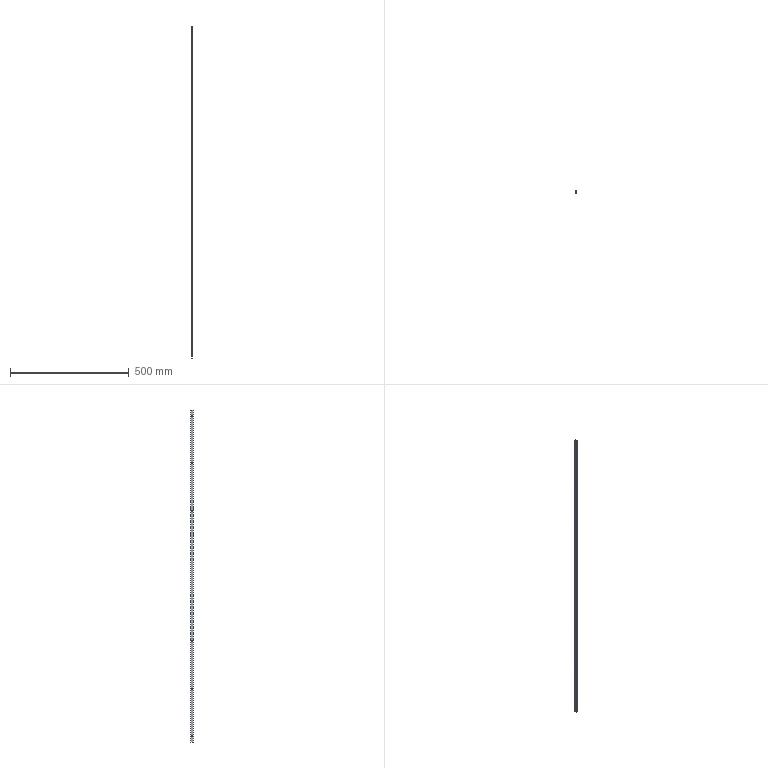Component | SolidWorks | GroundingSystem-1_GroundingCopperBar-1 | 1 solid | 18 faces | box 4 x 12 x 1400 mm | volume 66952 mm3 | cylinder 12 | plane 6 | commonest cylinder face diameters 3.3 x8 4.2 x4
STEP:
#1=COLOUR_RGB('',0.7922,0.8196,0.9333);
#2=FILL_AREA_STYLE_COLOUR('',#1);
#3=FILL_AREA_STYLE('',(#2));
#4=SURFACE_STYLE_FILL_AREA(#3);
#5=SURFACE_SIDE_STYLE('',(#4));
#6=SURFACE_STYLE_USAGE(.BOTH.,#5);
#7=PRESENTATION_STYLE_ASSIGNMENT((#6));
#8=CARTESIAN_POINT('',(10.505,-0.4112,58.688));
#9=VERTEX_POINT('',#8);
#10=CARTESIAN_POINT('',(10.505,-0.4112,58.853));
#11=VERTEX_POINT('',#10);
#12=CARTESIAN_POINT('',(10.505,-0.4112,58.771));
#13=DIRECTION('',(1.,0.,-0.));
#14=DIRECTION('',(0.,0.,1.));
#15=AXIS2_PLACEMENT_3D('',#12,#13,#14);
#16=CIRCLE('',#15,0.08268);
#17=EDGE_CURVE('',#9,#11,#16,.T.);
#18=ORIENTED_EDGE('',*,*,#17,.T.);
#19=CARTESIAN_POINT('',(10.348,-0.4112,58.853));
#20=VERTEX_POINT('',#19);
#21=CARTESIAN_POINT('',(10.348,-0.4112,58.853));
#22=DIRECTION('',(-1.,-0.,0.));
#23=VECTOR('',#22,39.37);
#24=LINE('',#21,#23);
#25=EDGE_CURVE('',#11,#20,#24,.T.);
#26=ORIENTED_EDGE('',*,*,#25,.T.);
#27=CARTESIAN_POINT('',(10.348,-0.4112,58.688));
#28=VERTEX_POINT('',#27);
#29=CARTESIAN_POINT('',(10.348,-0.4112,58.771));
#30=DIRECTION('',(-1.,-0.,0.));
#31=DIRECTION('',(0.,-0.,-1.));
#32=AXIS2_PLACEMENT_3D('',#29,#30,#31);
#33=CIRCLE('',#32,0.08268);
#34=EDGE_CURVE('',#20,#28,#33,.T.);
#35=ORIENTED_EDGE('',*,*,#34,.T.);
#36=CARTESIAN_POINT('',(10.348,-0.4112,58.688));
#37=DIRECTION('',(-1.,-0.,0.));
#38=VECTOR('',#37,39.37);
#39=LINE('',#36,#38);
#40=EDGE_CURVE('',#9,#28,#39,.T.);
#41=ORIENTED_EDGE('',*,*,#40,.F.);
#42=EDGE_LOOP('',(#18,#26,#35,#41));
#43=FACE_OUTER_BOUND('',#42,.T.);
#44=CARTESIAN_POINT('',(10.348,-0.4112,58.771));
#45=DIRECTION('',(-1.,-0.,0.));
#46=DIRECTION('',(0.,-0.,-1.));
#47=AXIS2_PLACEMENT_3D('',#44,#45,#46);
#48=CYLINDRICAL_SURFACE('',#47,0.08268);
#49=ADVANCED_FACE('',(#43),#48,.F.);
#50=CARTESIAN_POINT('',(10.505,-0.4112,5.538));
#51=VERTEX_POINT('',#50);
#52=CARTESIAN_POINT('',(10.505,-0.4112,5.704));
#53=VERTEX_POINT('',#52);
#54=CARTESIAN_POINT('',(10.505,-0.4112,5.621));
#55=DIRECTION('',(1.,0.,-0.));
#56=DIRECTION('',(0.,0.,1.));
#57=AXIS2_PLACEMENT_3D('',#54,#55,#56);
#58=CIRCLE('',#57,0.08268);
#59=EDGE_CURVE('',#51,#53,#58,.T.);
#60=ORIENTED_EDGE('',*,*,#59,.T.);
#61=CARTESIAN_POINT('',(10.348,-0.4112,5.704));
#62=VERTEX_POINT('',#61);
#63=CARTESIAN_POINT('',(10.348,-0.4112,5.704));
#64=DIRECTION('',(-1.,-0.,0.));
#65=VECTOR('',#64,39.37);
#66=LINE('',#63,#65);
#67=EDGE_CURVE('',#53,#62,#66,.T.);
#68=ORIENTED_EDGE('',*,*,#67,.T.);
#69=CARTESIAN_POINT('',(10.348,-0.4112,5.538));
#70=VERTEX_POINT('',#69);
#71=CARTESIAN_POINT('',(10.348,-0.4112,5.621));
#72=DIRECTION('',(-1.,-0.,0.));
#73=DIRECTION('',(0.,-0.,-1.));
#74=AXIS2_PLACEMENT_3D('',#71,#72,#73);
#75=CIRCLE('',#74,0.08268);
#76=EDGE_CURVE('',#62,#70,#75,.T.);
#77=ORIENTED_EDGE('',*,*,#76,.T.);
#78=CARTESIAN_POINT('',(10.348,-0.4112,5.538));
#79=DIRECTION('',(-1.,-0.,0.));
#80=VECTOR('',#79,39.37);
#81=LINE('',#78,#80);
#82=EDGE_CURVE('',#51,#70,#81,.T.);
#83=ORIENTED_EDGE('',*,*,#82,.F.);
#84=EDGE_LOOP('',(#60,#68,#77,#83));
#85=FACE_OUTER_BOUND('',#84,.T.);
#86=CARTESIAN_POINT('',(10.348,-0.4112,5.621));
#87=DIRECTION('',(-1.,-0.,0.));
#88=DIRECTION('',(0.,-0.,-1.));
#89=AXIS2_PLACEMENT_3D('',#86,#87,#88);
#90=CYLINDRICAL_SURFACE('',#89,0.08268);
#91=ADVANCED_FACE('',(#85),#90,.F.);
#92=CARTESIAN_POINT('',(10.505,-0.4112,50.832));
#93=VERTEX_POINT('',#92);
#94=CARTESIAN_POINT('',(10.505,-0.4112,50.962));
#95=VERTEX_POINT('',#94);
#96=CARTESIAN_POINT('',(10.505,-0.4112,50.897));
#97=DIRECTION('',(1.,0.,-0.));
#98=DIRECTION('',(0.,0.,1.));
#99=AXIS2_PLACEMENT_3D('',#96,#97,#98);
#100=CIRCLE('',#99,0.06496);
#101=EDGE_CURVE('',#93,#95,#100,.T.);
#102=ORIENTED_EDGE('',*,*,#101,.T.);
#103=CARTESIAN_POINT('',(10.348,-0.4112,50.962));
#104=VERTEX_POINT('',#103);
#105=CARTESIAN_POINT('',(10.348,-0.4112,50.962));
#106=DIRECTION('',(-1.,-0.,0.));
#107=VECTOR('',#106,39.37);
#108=LINE('',#105,#107);
#109=EDGE_CURVE('',#95,#104,#108,.T.);
#110=ORIENTED_EDGE('',*,*,#109,.T.);
#111=CARTESIAN_POINT('',(10.348,-0.4112,50.832));
#112=VERTEX_POINT('',#111);
#113=CARTESIAN_POINT('',(10.348,-0.4112,50.897));
#114=DIRECTION('',(-1.,-0.,0.));
#115=DIRECTION('',(0.,-0.,-1.));
#116=AXIS2_PLACEMENT_3D('',#113,#114,#115);
#117=CIRCLE('',#116,0.06496);
#118=EDGE_CURVE('',#104,#112,#117,.T.);
#119=ORIENTED_EDGE('',*,*,#118,.T.);
#120=CARTESIAN_POINT('',(10.348,-0.4112,50.832));
#121=DIRECTION('',(-1.,-0.,0.));
#122=VECTOR('',#121,39.37);
#123=LINE('',#120,#122);
#124=EDGE_CURVE('',#93,#112,#123,.T.);
#125=ORIENTED_EDGE('',*,*,#124,.F.);
#126=EDGE_LOOP('',(#102,#110,#119,#125));
#127=FACE_OUTER_BOUND('',#126,.T.);
#128=CARTESIAN_POINT('',(10.348,-0.4112,50.897));
#129=DIRECTION('',(-1.,-0.,0.));
#130=DIRECTION('',(0.,-0.,-1.));
#131=AXIS2_PLACEMENT_3D('',#128,#129,#130);
#132=CYLINDRICAL_SURFACE('',#131,0.06496);
#133=ADVANCED_FACE('',(#127),#132,.F.);
#134=CARTESIAN_POINT('',(10.505,-0.4112,42.958));
#135=VERTEX_POINT('',#134);
#136=CARTESIAN_POINT('',(10.505,-0.4112,43.088));
#137=VERTEX_POINT('',#136);
#138=CARTESIAN_POINT('',(10.505,-0.4112,43.023));
#139=DIRECTION('',(1.,0.,-0.));
#140=DIRECTION('',(0.,0.,1.));
#141=AXIS2_PLACEMENT_3D('',#138,#139,#140);
#142=CIRCLE('',#141,0.06496);
#143=EDGE_CURVE('',#135,#137,#142,.T.);
#144=ORIENTED_EDGE('',*,*,#143,.T.);
#145=CARTESIAN_POINT('',(10.348,-0.4112,43.088));
#146=VERTEX_POINT('',#145);
#147=CARTESIAN_POINT('',(10.348,-0.4112,43.088));
#148=DIRECTION('',(-1.,-0.,0.));
#149=VECTOR('',#148,39.37);
#150=LINE('',#147,#149);
#151=EDGE_CURVE('',#137,#146,#150,.T.);
#152=ORIENTED_EDGE('',*,*,#151,.T.);
#153=CARTESIAN_POINT('',(10.348,-0.4112,42.958));
#154=VERTEX_POINT('',#153);
#155=CARTESIAN_POINT('',(10.348,-0.4112,43.023));
#156=DIRECTION('',(-1.,-0.,0.));
#157=DIRECTION('',(0.,-0.,-1.));
#158=AXIS2_PLACEMENT_3D('',#155,#156,#157);
#159=CIRCLE('',#158,0.06496);
#160=EDGE_CURVE('',#146,#154,#159,.T.);
#161=ORIENTED_EDGE('',*,*,#160,.T.);
#162=CARTESIAN_POINT('',(10.348,-0.4112,42.958));
#163=DIRECTION('',(-1.,-0.,0.));
#164=VECTOR('',#163,39.37);
#165=LINE('',#162,#164);
#166=EDGE_CURVE('',#135,#154,#165,.T.);
#167=ORIENTED_EDGE('',*,*,#166,.F.);
#168=EDGE_LOOP('',(#144,#152,#161,#167));
#169=FACE_OUTER_BOUND('',#168,.T.);
#170=CARTESIAN_POINT('',(10.348,-0.4112,43.023));
#171=DIRECTION('',(-1.,-0.,0.));
#172=DIRECTION('',(0.,-0.,-1.));
#173=AXIS2_PLACEMENT_3D('',#170,#171,#172);
#174=CYLINDRICAL_SURFACE('',#173,0.06496);
#175=ADVANCED_FACE('',(#169),#174,.F.);
#176=CARTESIAN_POINT('',(10.505,-0.4112,13.43));
#177=VERTEX_POINT('',#176);
#178=CARTESIAN_POINT('',(10.505,-0.4112,13.56));
#179=VERTEX_POINT('',#178);
#180=CARTESIAN_POINT('',(10.505,-0.4112,13.495));
#181=DIRECTION('',(1.,0.,-0.));
#182=DIRECTION('',(0.,0.,1.));
#183=AXIS2_PLACEMENT_3D('',#180,#181,#182);
#184=CIRCLE('',#183,0.06496);
#185=EDGE_CURVE('',#177,#179,#184,.T.);
#186=ORIENTED_EDGE('',*,*,#185,.T.);
#187=CARTESIAN_POINT('',(10.348,-0.4112,13.56));
#188=VERTEX_POINT('',#187);
#189=CARTESIAN_POINT('',(10.348,-0.4112,13.56));
#190=DIRECTION('',(-1.,-0.,0.));
#191=VECTOR('',#190,39.37);
#192=LINE('',#189,#191);
#193=EDGE_CURVE('',#179,#188,#192,.T.);
#194=ORIENTED_EDGE('',*,*,#193,.T.);
#195=CARTESIAN_POINT('',(10.348,-0.4112,13.43));
#196=VERTEX_POINT('',#195);
#197=CARTESIAN_POINT('',(10.348,-0.4112,13.495));
#198=DIRECTION('',(-1.,-0.,0.));
#199=DIRECTION('',(0.,-0.,-1.));
#200=AXIS2_PLACEMENT_3D('',#197,#198,#199);
#201=CIRCLE('',#200,0.06496);
#202=EDGE_CURVE('',#188,#196,#201,.T.);
#203=ORIENTED_EDGE('',*,*,#202,.T.);
#204=CARTESIAN_POINT('',(10.348,-0.4112,13.43));
#205=DIRECTION('',(-1.,-0.,0.));
#206=VECTOR('',#205,39.37);
#207=LINE('',#204,#206);
#208=EDGE_CURVE('',#177,#196,#207,.T.);
#209=ORIENTED_EDGE('',*,*,#208,.F.);
#210=EDGE_LOOP('',(#186,#194,#203,#209));
#211=FACE_OUTER_BOUND('',#210,.T.);
#212=CARTESIAN_POINT('',(10.348,-0.4112,13.495));
#213=DIRECTION('',(-1.,-0.,0.));
#214=DIRECTION('',(0.,-0.,-1.));
#215=AXIS2_PLACEMENT_3D('',#212,#213,#214);
#216=CYLINDRICAL_SURFACE('',#215,0.06496);
#217=ADVANCED_FACE('',(#211),#216,.F.);
#218=CARTESIAN_POINT('',(10.505,-0.4112,21.304));
#219=VERTEX_POINT('',#218);
#220=CARTESIAN_POINT('',(10.505,-0.4112,21.434));
#221=VERTEX_POINT('',#220);
#222=CARTESIAN_POINT('',(10.505,-0.4112,21.369));
#223=DIRECTION('',(1.,0.,-0.));
#224=DIRECTION('',(0.,0.,1.));
#225=AXIS2_PLACEMENT_3D('',#222,#223,#224);
#226=CIRCLE('',#225,0.06496);
#227=EDGE_CURVE('',#219,#221,#226,.T.);
#228=ORIENTED_EDGE('',*,*,#227,.T.);
#229=CARTESIAN_POINT('',(10.348,-0.4112,21.434));
#230=VERTEX_POINT('',#229);
#231=CARTESIAN_POINT('',(10.348,-0.4112,21.434));
#232=DIRECTION('',(-1.,-0.,0.));
#233=VECTOR('',#232,39.37);
#234=LINE('',#231,#233);
#235=EDGE_CURVE('',#221,#230,#234,.T.);
#236=ORIENTED_EDGE('',*,*,#235,.T.);
#237=CARTESIAN_POINT('',(10.348,-0.4112,21.304));
#238=VERTEX_POINT('',#237);
#239=CARTESIAN_POINT('',(10.348,-0.4112,21.369));
#240=DIRECTION('',(-1.,-0.,0.));
#241=DIRECTION('',(0.,-0.,-1.));
#242=AXIS2_PLACEMENT_3D('',#239,#240,#241);
#243=CIRCLE('',#242,0.06496);
#244=EDGE_CURVE('',#230,#238,#243,.T.);
#245=ORIENTED_EDGE('',*,*,#244,.T.);
#246=CARTESIAN_POINT('',(10.348,-0.4112,21.304));
#247=DIRECTION('',(-1.,-0.,0.));
#248=VECTOR('',#247,39.37);
#249=LINE('',#246,#248);
#250=EDGE_CURVE('',#219,#238,#249,.T.);
#251=ORIENTED_EDGE('',*,*,#250,.F.);
#252=EDGE_LOOP('',(#228,#236,#245,#251));
#253=FACE_OUTER_BOUND('',#252,.T.);
#254=CARTESIAN_POINT('',(10.348,-0.4112,21.369));
#255=DIRECTION('',(-1.,-0.,0.));
#256=DIRECTION('',(0.,-0.,-1.));
#257=AXIS2_PLACEMENT_3D('',#254,#255,#256);
#258=CYLINDRICAL_SURFACE('',#257,0.06496);
#259=ADVANCED_FACE('',(#253),#258,.F.);
#260=CARTESIAN_POINT('',(10.348,-0.175,4.637));
#261=VERTEX_POINT('',#260);
#262=CARTESIAN_POINT('',(10.348,-0.6474,4.637));
#263=VERTEX_POINT('',#262);
#264=CARTESIAN_POINT('',(10.348,-0.175,4.637));
#265=DIRECTION('',(0.,-1.,0.));
#266=VECTOR('',#265,39.37);
#267=LINE('',#264,#266);
#268=EDGE_CURVE('',#261,#263,#267,.T.);
#269=ORIENTED_EDGE('',*,*,#268,.F.);
#270=CARTESIAN_POINT('',(10.505,-0.175,4.637));
#271=VERTEX_POINT('',#270);
#272=CARTESIAN_POINT('',(10.505,-0.175,4.637));
#273=DIRECTION('',(-1.,-0.,0.));
#274=VECTOR('',#273,39.37);
#275=LINE('',#272,#274);
#276=EDGE_CURVE('',#271,#261,#275,.T.);
#277=ORIENTED_EDGE('',*,*,#276,.F.);
#278=CARTESIAN_POINT('',(10.505,-0.6474,4.637));
#279=VERTEX_POINT('',#278);
#280=CARTESIAN_POINT('',(10.505,-0.175,4.637));
#281=DIRECTION('',(0.,-1.,0.));
#282=VECTOR('',#281,39.37);
#283=LINE('',#280,#282);
#284=EDGE_CURVE('',#271,#279,#283,.T.);
#285=ORIENTED_EDGE('',*,*,#284,.T.);
#286=CARTESIAN_POINT('',(10.505,-0.6474,4.637));
#287=DIRECTION('',(-1.,-0.,0.));
#288=VECTOR('',#287,39.37);
#289=LINE('',#286,#288);
#290=EDGE_CURVE('',#279,#263,#289,.T.);
#291=ORIENTED_EDGE('',*,*,#290,.T.);
#292=EDGE_LOOP('',(#269,#277,#285,#291));
#293=FACE_OUTER_BOUND('',#292,.T.);
#294=CARTESIAN_POINT('',(10.505,-0.175,4.637));
#295=DIRECTION('',(-0.,-0.,-1.));
#296=DIRECTION('',(1.,0.,-0.));
#297=AXIS2_PLACEMENT_3D('',#294,#295,#296);
#298=PLANE('',#297);
#299=ADVANCED_FACE('',(#293),#298,.T.);
#300=CARTESIAN_POINT('',(10.348,-0.175,59.755));
#301=VERTEX_POINT('',#300);
#302=CARTESIAN_POINT('',(10.348,-0.175,59.755));
#303=DIRECTION('',(-0.,-0.,-1.));
#304=VECTOR('',#303,39.37);
#305=LINE('',#302,#304);
#306=EDGE_CURVE('',#301,#261,#305,.T.);
#307=ORIENTED_EDGE('',*,*,#306,.F.);
#308=CARTESIAN_POINT('',(10.505,-0.175,59.755));
#309=VERTEX_POINT('',#308);
#310=CARTESIAN_POINT('',(10.505,-0.175,59.755));
#311=DIRECTION('',(-1.,-0.,0.));
#312=VECTOR('',#311,39.37);
#313=LINE('',#310,#312);
#314=EDGE_CURVE('',#309,#301,#313,.T.);
#315=ORIENTED_EDGE('',*,*,#314,.F.);
#316=CARTESIAN_POINT('',(10.505,-0.175,59.755));
#317=DIRECTION('',(-0.,-0.,-1.));
#318=VECTOR('',#317,39.37);
#319=LINE('',#316,#318);
#320=EDGE_CURVE('',#309,#271,#319,.T.);
#321=ORIENTED_EDGE('',*,*,#320,.T.);
#322=ORIENTED_EDGE('',*,*,#276,.T.);
#323=EDGE_LOOP('',(#307,#315,#321,#322));
#324=FACE_OUTER_BOUND('',#323,.T.);
#325=CARTESIAN_POINT('',(10.505,-0.175,59.755));
#326=DIRECTION('',(-0.,1.,-0.));
#327=DIRECTION('',(1.,0.,-0.));
#328=AXIS2_PLACEMENT_3D('',#325,#326,#327);
#329=PLANE('',#328);
#330=ADVANCED_FACE('',(#324),#329,.T.);
#331=CARTESIAN_POINT('',(10.348,-0.6474,59.755));
#332=VERTEX_POINT('',#331);
#333=CARTESIAN_POINT('',(10.348,-0.175,59.755));
#334=DIRECTION('',(-0.,1.,-0.));
#335=VECTOR('',#334,39.37);
#336=LINE('',#333,#335);
#337=EDGE_CURVE('',#332,#301,#336,.T.);
#338=ORIENTED_EDGE('',*,*,#337,.F.);
#339=CARTESIAN_POINT('',(10.505,-0.6474,59.755));
#340=VERTEX_POINT('',#339);
#341=CARTESIAN_POINT('',(10.505,-0.6474,59.755));
#342=DIRECTION('',(-1.,-0.,0.));
#343=VECTOR('',#342,39.37);
#344=LINE('',#341,#343);
#345=EDGE_CURVE('',#340,#332,#344,.T.);
#346=ORIENTED_EDGE('',*,*,#345,.F.);
#347=CARTESIAN_POINT('',(10.505,-0.175,59.755));
#348=DIRECTION('',(-0.,1.,-0.));
#349=VECTOR('',#348,39.37);
#350=LINE('',#347,#349);
#351=EDGE_CURVE('',#340,#309,#350,.T.);
#352=ORIENTED_EDGE('',*,*,#351,.T.);
#353=ORIENTED_EDGE('',*,*,#314,.T.);
#354=EDGE_LOOP('',(#338,#346,#352,#353));
#355=FACE_OUTER_BOUND('',#354,.T.);
#356=CARTESIAN_POINT('',(10.505,-0.175,59.755));
#357=DIRECTION('',(0.,0.,1.));
#358=DIRECTION('',(-1.,-0.,0.));
#359=AXIS2_PLACEMENT_3D('',#356,#357,#358);
#360=PLANE('',#359);
#361=ADVANCED_FACE('',(#355),#360,.T.);
#362=CARTESIAN_POINT('',(10.348,-0.6474,59.755));
#363=DIRECTION('',(0.,0.,1.));
#364=VECTOR('',#363,39.37);
#365=LINE('',#362,#364);
#366=EDGE_CURVE('',#263,#332,#365,.T.);
#367=ORIENTED_EDGE('',*,*,#366,.F.);
#368=ORIENTED_EDGE('',*,*,#290,.F.);
#369=CARTESIAN_POINT('',(10.505,-0.6474,59.755));
#370=DIRECTION('',(0.,0.,1.));
#371=VECTOR('',#370,39.37);
#372=LINE('',#369,#371);
#373=EDGE_CURVE('',#279,#340,#372,.T.);
#374=ORIENTED_EDGE('',*,*,#373,.T.);
#375=ORIENTED_EDGE('',*,*,#345,.T.);
#376=EDGE_LOOP('',(#367,#368,#374,#375));
#377=FACE_OUTER_BOUND('',#376,.T.);
#378=CARTESIAN_POINT('',(10.505,-0.6474,59.755));
#379=DIRECTION('',(0.,-1.,0.));
#380=DIRECTION('',(-1.,-0.,0.));
#381=AXIS2_PLACEMENT_3D('',#378,#379,#380);
#382=PLANE('',#381);
#383=ADVANCED_FACE('',(#377),#382,.T.);
#384=ORIENTED_EDGE('',*,*,#17,.F.);
#385=CARTESIAN_POINT('',(10.505,-0.4112,58.771));
#386=DIRECTION('',(1.,0.,-0.));
#387=DIRECTION('',(0.,0.,1.));
#388=AXIS2_PLACEMENT_3D('',#385,#386,#387);
#389=CIRCLE('',#388,0.08268);
#390=EDGE_CURVE('',#11,#9,#389,.T.);
#391=ORIENTED_EDGE('',*,*,#390,.F.);
#392=EDGE_LOOP('',(#384,#391));
#393=FACE_BOUND('',#392,.T.);
#394=ORIENTED_EDGE('',*,*,#59,.F.);
#395=CARTESIAN_POINT('',(10.505,-0.4112,5.621));
#396=DIRECTION('',(1.,0.,-0.));
#397=DIRECTION('',(0.,0.,1.));
#398=AXIS2_PLACEMENT_3D('',#395,#396,#397);
#399=CIRCLE('',#398,0.08268);
#400=EDGE_CURVE('',#53,#51,#399,.T.);
#401=ORIENTED_EDGE('',*,*,#400,.F.);
#402=EDGE_LOOP('',(#394,#401));
#403=FACE_BOUND('',#402,.T.);
#404=ORIENTED_EDGE('',*,*,#101,.F.);
#405=CARTESIAN_POINT('',(10.505,-0.4112,50.897));
#406=DIRECTION('',(1.,0.,-0.));
#407=DIRECTION('',(0.,0.,1.));
#408=AXIS2_PLACEMENT_3D('',#405,#406,#407);
#409=CIRCLE('',#408,0.06496);
#410=EDGE_CURVE('',#95,#93,#409,.T.);
#411=ORIENTED_EDGE('',*,*,#410,.F.);
#412=EDGE_LOOP('',(#404,#411));
#413=FACE_BOUND('',#412,.T.);
#414=ORIENTED_EDGE('',*,*,#143,.F.);
#415=CARTESIAN_POINT('',(10.505,-0.4112,43.023));
#416=DIRECTION('',(1.,0.,-0.));
#417=DIRECTION('',(0.,0.,1.));
#418=AXIS2_PLACEMENT_3D('',#415,#416,#417);
#419=CIRCLE('',#418,0.06496);
#420=EDGE_CURVE('',#137,#135,#419,.T.);
#421=ORIENTED_EDGE('',*,*,#420,.F.);
#422=EDGE_LOOP('',(#414,#421));
#423=FACE_BOUND('',#422,.T.);
#424=ORIENTED_EDGE('',*,*,#185,.F.);
#425=CARTESIAN_POINT('',(10.505,-0.4112,13.495));
#426=DIRECTION('',(1.,0.,-0.));
#427=DIRECTION('',(0.,0.,1.));
#428=AXIS2_PLACEMENT_3D('',#425,#426,#427);
#429=CIRCLE('',#428,0.06496);
#430=EDGE_CURVE('',#179,#177,#429,.T.);
#431=ORIENTED_EDGE('',*,*,#430,.F.);
#432=EDGE_LOOP('',(#424,#431));
#433=FACE_BOUND('',#432,.T.);
#434=ORIENTED_EDGE('',*,*,#227,.F.);
#435=CARTESIAN_POINT('',(10.505,-0.4112,21.369));
#436=DIRECTION('',(1.,0.,-0.));
#437=DIRECTION('',(0.,0.,1.));
#438=AXIS2_PLACEMENT_3D('',#435,#436,#437);
#439=CIRCLE('',#438,0.06496);
#440=EDGE_CURVE('',#221,#219,#439,.T.);
#441=ORIENTED_EDGE('',*,*,#440,.F.);
#442=EDGE_LOOP('',(#434,#441));
#443=FACE_BOUND('',#442,.T.);
#444=ORIENTED_EDGE('',*,*,#284,.F.);
#445=ORIENTED_EDGE('',*,*,#320,.F.);
#446=ORIENTED_EDGE('',*,*,#351,.F.);
#447=ORIENTED_EDGE('',*,*,#373,.F.);
#448=EDGE_LOOP('',(#444,#445,#446,#447));
#449=FACE_OUTER_BOUND('',#448,.T.);
#450=CARTESIAN_POINT('',(10.505,-0.6474,4.637));
#451=DIRECTION('',(1.,0.,-0.));
#452=DIRECTION('',(0.,0.,1.));
#453=AXIS2_PLACEMENT_3D('',#450,#451,#452);
#454=PLANE('',#453);
#455=ADVANCED_FACE('',(#393,#403,#413,#423,#433,#443,#449),#454,.T.);
#456=CARTESIAN_POINT('',(10.348,-0.4112,58.771));
#457=DIRECTION('',(-1.,-0.,0.));
#458=DIRECTION('',(0.,-0.,-1.));
#459=AXIS2_PLACEMENT_3D('',#456,#457,#458);
#460=CIRCLE('',#459,0.08268);
#461=EDGE_CURVE('',#28,#20,#460,.T.);
#462=ORIENTED_EDGE('',*,*,#461,.F.);
#463=ORIENTED_EDGE('',*,*,#34,.F.);
#464=EDGE_LOOP('',(#462,#463));
#465=FACE_BOUND('',#464,.T.);
#466=CARTESIAN_POINT('',(10.348,-0.4112,5.621));
#467=DIRECTION('',(-1.,-0.,0.));
#468=DIRECTION('',(0.,-0.,-1.));
#469=AXIS2_PLACEMENT_3D('',#466,#467,#468);
#470=CIRCLE('',#469,0.08268);
#471=EDGE_CURVE('',#70,#62,#470,.T.);
#472=ORIENTED_EDGE('',*,*,#471,.F.);
#473=ORIENTED_EDGE('',*,*,#76,.F.);
#474=EDGE_LOOP('',(#472,#473));
#475=FACE_BOUND('',#474,.T.);
#476=CARTESIAN_POINT('',(10.348,-0.4112,50.897));
#477=DIRECTION('',(-1.,-0.,0.));
#478=DIRECTION('',(0.,-0.,-1.));
#479=AXIS2_PLACEMENT_3D('',#476,#477,#478);
#480=CIRCLE('',#479,0.06496);
#481=EDGE_CURVE('',#112,#104,#480,.T.);
#482=ORIENTED_EDGE('',*,*,#481,.F.);
#483=ORIENTED_EDGE('',*,*,#118,.F.);
#484=EDGE_LOOP('',(#482,#483));
#485=FACE_BOUND('',#484,.T.);
#486=CARTESIAN_POINT('',(10.348,-0.4112,43.023));
#487=DIRECTION('',(-1.,-0.,0.));
#488=DIRECTION('',(0.,-0.,-1.));
#489=AXIS2_PLACEMENT_3D('',#486,#487,#488);
#490=CIRCLE('',#489,0.06496);
#491=EDGE_CURVE('',#154,#146,#490,.T.);
#492=ORIENTED_EDGE('',*,*,#491,.F.);
#493=ORIENTED_EDGE('',*,*,#160,.F.);
#494=EDGE_LOOP('',(#492,#493));
#495=FACE_BOUND('',#494,.T.);
#496=CARTESIAN_POINT('',(10.348,-0.4112,13.495));
#497=DIRECTION('',(-1.,-0.,0.));
#498=DIRECTION('',(0.,-0.,-1.));
#499=AXIS2_PLACEMENT_3D('',#496,#497,#498);
#500=CIRCLE('',#499,0.06496);
#501=EDGE_CURVE('',#196,#188,#500,.T.);
#502=ORIENTED_EDGE('',*,*,#501,.F.);
#503=ORIENTED_EDGE('',*,*,#202,.F.);
#504=EDGE_LOOP('',(#502,#503));
#505=FACE_BOUND('',#504,.T.);
#506=CARTESIAN_POINT('',(10.348,-0.4112,21.369));
#507=DIRECTION('',(-1.,-0.,0.));
#508=DIRECTION('',(0.,-0.,-1.));
#509=AXIS2_PLACEMENT_3D('',#506,#507,#508);
#510=CIRCLE('',#509,0.06496);
#511=EDGE_CURVE('',#238,#230,#510,.T.);
#512=ORIENTED_EDGE('',*,*,#511,.F.);
#513=ORIENTED_EDGE('',*,*,#244,.F.);
#514=EDGE_LOOP('',(#512,#513));
#515=FACE_BOUND('',#514,.T.);
#516=ORIENTED_EDGE('',*,*,#268,.T.);
#517=ORIENTED_EDGE('',*,*,#366,.T.);
#518=ORIENTED_EDGE('',*,*,#337,.T.);
#519=ORIENTED_EDGE('',*,*,#306,.T.);
#520=EDGE_LOOP('',(#516,#517,#518,#519));
#521=FACE_OUTER_BOUND('',#520,.T.);
#522=CARTESIAN_POINT('',(10.348,-0.6474,4.637));
#523=DIRECTION('',(1.,0.,-0.));
#524=DIRECTION('',(0.,0.,1.));
#525=AXIS2_PLACEMENT_3D('',#522,#523,#524);
#526=PLANE('',#525);
#527=ADVANCED_FACE('',(#465,#475,#485,#495,#505,#515,#521),#526,.F.);
#528=ORIENTED_EDGE('',*,*,#235,.F.);
#529=ORIENTED_EDGE('',*,*,#440,.T.);
#530=ORIENTED_EDGE('',*,*,#250,.T.);
#531=ORIENTED_EDGE('',*,*,#511,.T.);
#532=EDGE_LOOP('',(#528,#529,#530,#531));
#533=FACE_OUTER_BOUND('',#532,.T.);
#534=CARTESIAN_POINT('',(10.348,-0.4112,21.369));
#535=DIRECTION('',(-1.,-0.,0.));
#536=DIRECTION('',(0.,-0.,-1.));
#537=AXIS2_PLACEMENT_3D('',#534,#535,#536);
#538=CYLINDRICAL_SURFACE('',#537,0.06496);
#539=ADVANCED_FACE('',(#533),#538,.F.);
#540=ORIENTED_EDGE('',*,*,#193,.F.);
#541=ORIENTED_EDGE('',*,*,#430,.T.);
#542=ORIENTED_EDGE('',*,*,#208,.T.);
#543=ORIENTED_EDGE('',*,*,#501,.T.);
#544=EDGE_LOOP('',(#540,#541,#542,#543));
#545=FACE_OUTER_BOUND('',#544,.T.);
#546=CARTESIAN_POINT('',(10.348,-0.4112,13.495));
#547=DIRECTION('',(-1.,-0.,0.));
#548=DIRECTION('',(0.,-0.,-1.));
#549=AXIS2_PLACEMENT_3D('',#546,#547,#548);
#550=CYLINDRICAL_SURFACE('',#549,0.06496);
#551=ADVANCED_FACE('',(#545),#550,.F.);
#552=ORIENTED_EDGE('',*,*,#151,.F.);
#553=ORIENTED_EDGE('',*,*,#420,.T.);
#554=ORIENTED_EDGE('',*,*,#166,.T.);
#555=ORIENTED_EDGE('',*,*,#491,.T.);
#556=EDGE_LOOP('',(#552,#553,#554,#555));
#557=FACE_OUTER_BOUND('',#556,.T.);
#558=CARTESIAN_POINT('',(10.348,-0.4112,43.023));
#559=DIRECTION('',(-1.,-0.,0.));
#560=DIRECTION('',(0.,-0.,-1.));
#561=AXIS2_PLACEMENT_3D('',#558,#559,#560);
#562=CYLINDRICAL_SURFACE('',#561,0.06496);
#563=ADVANCED_FACE('',(#557),#562,.F.);
#564=ORIENTED_EDGE('',*,*,#109,.F.);
#565=ORIENTED_EDGE('',*,*,#410,.T.);
#566=ORIENTED_EDGE('',*,*,#124,.T.);
#567=ORIENTED_EDGE('',*,*,#481,.T.);
#568=EDGE_LOOP('',(#564,#565,#566,#567));
#569=FACE_OUTER_BOUND('',#568,.T.);
#570=CARTESIAN_POINT('',(10.348,-0.4112,50.897));
#571=DIRECTION('',(-1.,-0.,0.));
#572=DIRECTION('',(0.,-0.,-1.));
#573=AXIS2_PLACEMENT_3D('',#570,#571,#572);
#574=CYLINDRICAL_SURFACE('',#573,0.06496);
#575=ADVANCED_FACE('',(#569),#574,.F.);
#576=ORIENTED_EDGE('',*,*,#67,.F.);
#577=ORIENTED_EDGE('',*,*,#400,.T.);
#578=ORIENTED_EDGE('',*,*,#82,.T.);
#579=ORIENTED_EDGE('',*,*,#471,.T.);
#580=EDGE_LOOP('',(#576,#577,#578,#579));
#581=FACE_OUTER_BOUND('',#580,.T.);
#582=CARTESIAN_POINT('',(10.348,-0.4112,5.621));
#583=DIRECTION('',(-1.,-0.,0.));
#584=DIRECTION('',(0.,-0.,-1.));
#585=AXIS2_PLACEMENT_3D('',#582,#583,#584);
#586=CYLINDRICAL_SURFACE('',#585,0.08268);
#587=ADVANCED_FACE('',(#581),#586,.F.);
#588=ORIENTED_EDGE('',*,*,#25,.F.);
#589=ORIENTED_EDGE('',*,*,#390,.T.);
#590=ORIENTED_EDGE('',*,*,#40,.T.);
#591=ORIENTED_EDGE('',*,*,#461,.T.);
#592=EDGE_LOOP('',(#588,#589,#590,#591));
#593=FACE_OUTER_BOUND('',#592,.T.);
#594=CARTESIAN_POINT('',(10.348,-0.4112,58.771));
#595=DIRECTION('',(-1.,-0.,0.));
#596=DIRECTION('',(0.,-0.,-1.));
#597=AXIS2_PLACEMENT_3D('',#594,#595,#596);
#598=CYLINDRICAL_SURFACE('',#597,0.08268);
#599=ADVANCED_FACE('',(#593),#598,.F.);
#600=CLOSED_SHELL('',(#49,#91,#133,#175,#217,#259,#299,#330,#361,#383,#455,#527,#539,#551,#563,#575,#587,#599));
#601=MANIFOLD_SOLID_BREP('',#600);
#602=STYLED_ITEM('',(#7),#601);
#603=(LENGTH_UNIT()NAMED_UNIT(*)SI_UNIT($,.METRE.));
#604=LENGTH_MEASURE_WITH_UNIT(LENGTH_MEASURE(0.0254),#603);
#605=DIMENSIONAL_EXPONENTS(1.,0.,0.,0.,0.,0.,0.);
#606=(CONVERSION_BASED_UNIT('',#604)LENGTH_UNIT()NAMED_UNIT(#605));
#607=UNCERTAINTY_MEASURE_WITH_UNIT(LENGTH_MEASURE(0.00001),#606,'','');
#608=(NAMED_UNIT(*)PLANE_ANGLE_UNIT()SI_UNIT($,.RADIAN.));
#609=(NAMED_UNIT(*)SI_UNIT($,.STERADIAN.)SOLID_ANGLE_UNIT());
#610=(GEOMETRIC_REPRESENTATION_CONTEXT(3)GLOBAL_UNCERTAINTY_ASSIGNED_CONTEXT((#607))GLOBAL_UNIT_ASSIGNED_CONTEXT((#606,#608,#609))REPRESENTATION_CONTEXT('',''));
#611=MECHANICAL_DESIGN_GEOMETRIC_PRESENTATION_REPRESENTATION('',(#602),#610);
#612=CARTESIAN_POINT('',(0.,0.,0.));
#613=DIRECTION('',(0.,0.,1.));
#614=DIRECTION('',(1.,0.,0.));
#615=AXIS2_PLACEMENT_3D('',#612,#613,#614);
#616=(LENGTH_UNIT()NAMED_UNIT(*)SI_UNIT($,.METRE.));
#617=LENGTH_MEASURE_WITH_UNIT(LENGTH_MEASURE(0.0254),#616);
#618=DIMENSIONAL_EXPONENTS(1.,0.,0.,0.,0.,0.,0.);
#619=(CONVERSION_BASED_UNIT('',#617)LENGTH_UNIT()NAMED_UNIT(#618));
#620=UNCERTAINTY_MEASURE_WITH_UNIT(LENGTH_MEASURE(0.00001),#619,'','');
#621=(NAMED_UNIT(*)PLANE_ANGLE_UNIT()SI_UNIT($,.RADIAN.));
#622=(NAMED_UNIT(*)SI_UNIT($,.STERADIAN.)SOLID_ANGLE_UNIT());
#623=(GEOMETRIC_REPRESENTATION_CONTEXT(3)GLOBAL_UNCERTAINTY_ASSIGNED_CONTEXT((#620))GLOBAL_UNIT_ASSIGNED_CONTEXT((#619,#621,#622))REPRESENTATION_CONTEXT('',''));
#624=ADVANCED_BREP_SHAPE_REPRESENTATION('',(#601,#615),#623);
#625=PRESENTATION_LAYER_ASSIGNMENT('','',(#602));